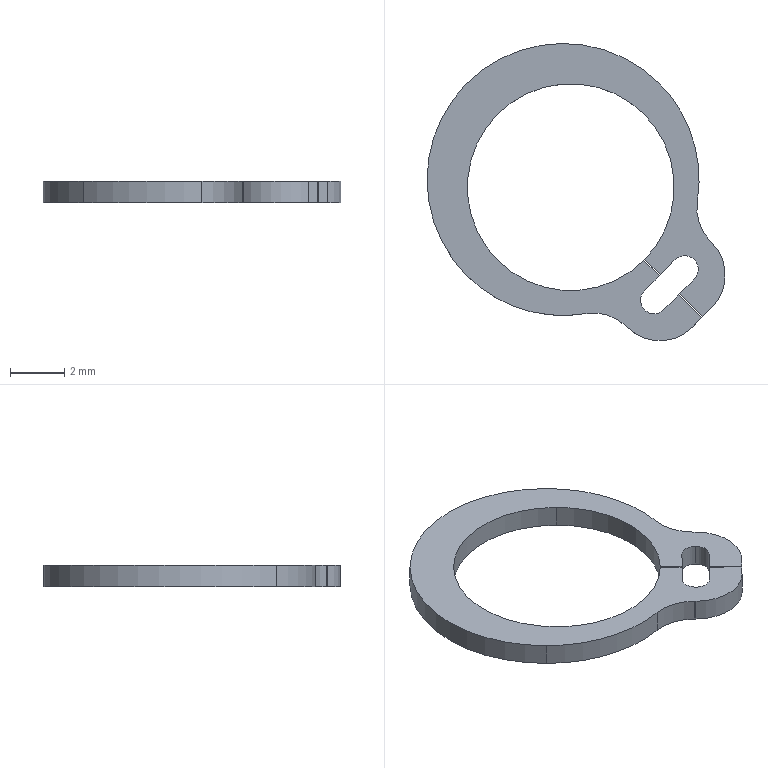Component | SolidWorks | RetainingRing~STWN8~MISUMI-1111-1 | 1 solid | 27 faces | volume 32 mm3 | plane 14 | cylinder 13 | commonest cylinder face diameters 3.4 x4 1 x3 7.6 x3 10 x3